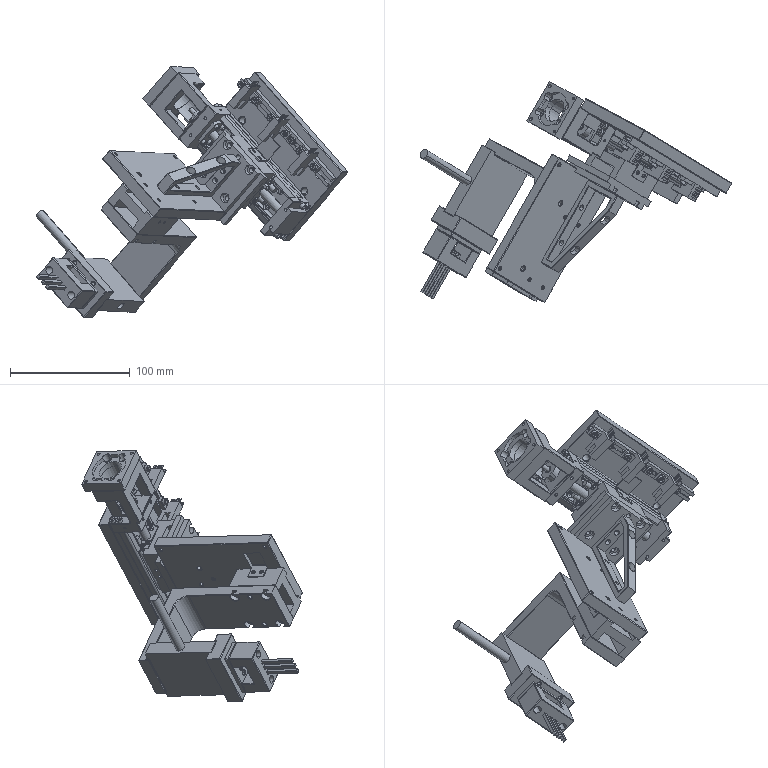Assembly | SolidWorks | mm | 37 component files | 37 solids | 2007 faces | box 260.89 x 184.6 x 210.11 mm | volume 491742 mm3 | plane 1154 | cylinder 578 | cone 238 | spline 35 | torus 2 | commonest cylinder face diameters 2.5 x74 3 x49 1 x41 4 x38 6.5 x36 3.4 x36 8 x30 3.5 x30
Bill of materials:
1z0-123 | 2 |  | Rectangular block with a raised strip along one top edge and a wide rectangular channel cut through the underside, leaving two end legs; four through holes on the top face and two small holes on one side face.
2z0-123 | 1 |  | L-shaped angle bracket: two flat legs at about 90 degrees with an inside fillet at the bend; each leg has two rows of three holes, and small rectangular notches along the edges.
3z0-123 | 1 |  | Rectangular block with a counterbored central through hole flanked by two smaller holes; one face has a longitudinal groove with a smaller hole and a larger bore, and there are small notches and a shallow rectangular slot.
4z0-123 | 1 |  | C-shaped block (rectangular block with a large rectangular notch cut from one side) with two large round holes and three square openings, shown rotated like diamonds, on the back face, plus smaller round holes on the arm faces.
5z0-123 | 1 |  | Flat rectangular plate with chamfered edges and five holes in a line: two smaller outer holes and three larger inner holes that appear stepped.
6z0-123 | 3 |  | Long square-section bar with a larger square head at one end; edges are chamfered and the head end appears to have a round bore.
7z0-123 | 1 |  | Thick rectangular plate with a scattered pattern of holes of several sizes on the main face, small holes near the corners, and a row of holes on one narrow edge face.
8z0-123 | 1 |  | Square plate with a stepped rebate along one edge, several counterbored holes, plain holes of various sizes, small edge notches, and two small rectangular blocks on the opposite face.
9z0-123 | 1 |  | Open triangular/trapezoidal frame made of rectangular-section members with a chamfered corner; the long sloped member has two large holes, and the other members have smaller holes.
GravitySensorZ0-123 | 1 |  | Rectangular block with a cylindrical rod sticking out from one narrow face, and round holes on two other side faces.
f2z0-123 | 1 |  | Thick square block with a large central through bore, surrounded by a pattern of smaller holes and corner holes; one face has stepped, lobed recesses around the bore.
KK40-100_8z0-123 | 1 |  | Long multi-body assembly: a square end block with a large bore and hole pattern, an open rectangular frame section with a cylindrical body inside, a long body with parallel round rods and a plate, and an end block showing several screw-head-like cylinders.
KK40-A1_1z0-123 | 1 |  | Compact rectangular block-like multi-body unit with parallel cylindrical rods running along its length, a top plate with recessed pads and holes, and pan-head cross-recess screws plus protruding round pins at the end faces.
CB3-6-0710z0-123 | 7 |  | Socket-head cap screw shape: cylindrical head with hexagonal socket recess and a plain cylindrical shank with chamfered end.
CBTN3-0710z0-123 | 6 |  | Hexagonal nut with central through bore and chamfered corners on one or both faces.
EE-SX672-0710z0-123 | 3 |  | U-shaped (slotted) housing with two parallel arms separated by a gap, a perpendicular mounting flange with two through holes, and a row of four thin flat pin-like tabs projecting from one end.
SENA34H-400-V50-W150-X250-Y350-N3.5-0710z0-123 | 1 |  | Long straight prismatic bar with a C/slotted channel cross-section and a small transverse hole near mid-length.
Part7z0-123 | 1 |  | Flat rectangular plate with a pattern of through holes of several sizes, including counterbored holes near corners and smaller holes.
ShadingPlateZ0-123 | 2 |  | Bent sheet-like angle bracket (L-shape) with a rounded bend; one leg has two round through holes, the other leg is plain.
ur3_15-0710z0-123 | 1 |  | Hollow thin-walled cylindrical sleeve with an axial split/overlapping seam, resembling a rolled or slotted tube.
Mates:
1. width | GravitySensorZ0-123-1 face at (-90.302, -65.883, 90.305) dir (-0.6119, 0.3716, 0.6982) | GravitySensorZ0-123-1 face at (-59.217, -84.759, 54.836) dir (0.6119, -0.3716, -0.6982) | 1z0-123-1 face at (-3.382, -95.961, 117.465) dir (0.6119, -0.3716, -0.6982) | 1z0-123-1 face at (-27.859, -81.098, 145.394) dir (-0.6119, 0.3716, 0.6982)
2. coincident | GravitySensorZ0-123-1 face at (-59.217, -84.759, 54.836) dir (-0.4977, -0.867, 0.02519) | 3z0-123-1 face at (-59.279, -84.726, 54.764) dir (0.4977, 0.867, -0.02519)
3. coincident | GravitySensorZ0-123-1 face at (-51.151, -52.012, 80.856) dir (0.6147, -0.3321, 0.7154) | 3z0-123-1 face at (-51.411, -88.977, 63.922) dir (-0.6147, 0.3321, -0.7154)
4. coincident | GravitySensorZ0-123-1 face at (-90.302, -65.883, 90.305) dir (-0.6119, 0.3716, 0.6982) | 3z0-123-1 face at (-94.655, -61.26, 84.03) dir (-0.6119, 0.3716, 0.6982)
5. width | 4z0-123-1 face at (-71.913, -121.978, 71.25) dir (0.6147, -0.3321, 0.7154) | 4z0-123-1 face at (-84.207, -115.336, 56.941) dir (-0.6147, 0.3321, -0.7154) | 3z0-123-1 face at (-94.655, -61.26, 84.03) dir (-0.6147, 0.3321, -0.7154) | 3z0-123-1 face at (-76.214, -71.223, 105.493) dir (0.6147, -0.3321, 0.7154)
6. width | 4z0-123-1 face at (-84.207, -115.336, 56.941) dir (0.6119, -0.3716, -0.6982) | 4z0-123-1 face at (-108.683, -100.473, 84.87) dir (-0.6119, 0.3716, 0.6982) | 3z0-123-1 face at (-94.655, -61.26, 84.03) dir (-0.6119, 0.3716, 0.6982) | 3z0-123-1 face at (-63.57, -80.136, 48.561) dir (0.6119, -0.3716, -0.6982)
7. coincident | 4z0-123-1 face at (-78.851, -91.285, 77.48) dir (0.4977, 0.867, -0.02519) | 5z0-123-1 face at (-78.851, -91.285, 77.48) dir (-0.4977, -0.867, 0.02519)
8. coincident | 4z0-123-1 face at (-84.207, -115.336, 56.941) dir (0.6119, -0.3716, -0.6982) | 5z0-123-1 face at (-58.475, -98.569, 70.57) dir (0.6119, -0.3716, -0.6982)
9. coincident | 4z0-123-1 face at (-84.207, -115.336, 56.941) dir (-0.6147, 0.3321, -0.7154) | 5z0-123-1 face at (-95.245, -77.065, 84.189) dir (-0.6147, 0.3321, -0.7154)
10. coincident | 3z0-123-1 face at (-76.86, -87.817, 77.38) dir (-0.4977, -0.867, 0.02519) | 5z0-123-1 face at (-76.86, -87.817, 77.38) dir (0.4977, 0.867, -0.02519)
11. coincident | 4z0-123-1 face at (-84.851, -102.083, 63.646) dir (0.4977, 0.867, -0.02519) | 6z0-123-1 face at (-88.495, -99.459, 81.972) dir (-0.4977, -0.867, 0.02519)
12. coincident | 6z0-123-1 face at (-108.403, -134.138, 82.98) dir (-0.4977, -0.867, 0.02519) | 6z0-123-2 face at (-104.732, -136.368, 78.79) dir (-0.4977, -0.867, 0.02519)
13. coincident | 6z0-123-1 face at (-108.403, -134.138, 82.98) dir (-0.4977, -0.867, 0.02519) | 6z0-123-3 face at (-101.06, -138.597, 74.601) dir (-0.4977, -0.867, 0.02519)
14. concentric | 5z0-123-1 face at (-77.855, -89.551, 77.43) dir (-0.4977, -0.867, 0.02519) r 2.1 | 6z0-123-2 face at (-83.828, -99.955, 77.732) dir (0.4977, 0.867, -0.02519) r 2.1
15. concentric | 5z0-123-1 face at (-74.184, -91.78, 73.241) dir (-0.4977, -0.867, 0.02519) r 2.1 | 6z0-123-3 face at (-80.156, -102.184, 73.543) dir (0.4977, 0.867, -0.02519) r 2.1
16. concentric | 6z0-123-1 face at (-87.499, -97.725, 81.922) dir (0.4977, 0.867, -0.02519) r 2.1 | ur3_15-0710z0-123-1 face at (-83.767, -91.223, 81.733) dir (-0.4977, -0.867, 0.02519) r 1.5
17. tangent | 6z0-123-1 face at (-87.499, -97.725, 81.922) dir (0.4977, 0.867, -0.02519) | ur3_15-0710z0-123-1 face at (-87.969, -97.077, 83.049) dir (1, 0, 0)
18. coincident | 7z0-123-1 face at (-0.3267, -18.072, 178.948) dir (0.4977, 0.867, -0.02519) | 8z0-123-1 face at (43.801, -43.838, 164.019) dir (-0.4977, -0.867, 0.02519)
19. coincident | 8z0-123-1 face at (42.307, -46.439, 164.094) dir (-0.4977, -0.867, 0.02519) | 9z0-123-1 face at (36.147, -43.316, 149.872) dir (0.4977, 0.867, -0.02519)
20. coincident | 7z0-123-1 face at (-0.1369, -82.082, 163.051) dir (0.6147, -0.3321, 0.7154) | 9z0-123-1 face at (-3.67, -112.674, 151.887) dir (-0.6147, 0.3321, -0.7154)
21. width | 9z0-123-1 face at (28.532, -84.637, 165.188) dir (0.6119, -0.3716, -0.6982) | 9z0-123-1 face at (22.413, -80.921, 172.17) dir (-0.6119, 0.3716, 0.6982) | 8z0-123-1 face at (37.941, -45.023, 126.572) dir (0.6119, -0.3716, -0.6982) | 8z0-123-1 face at (9.793, -27.93, 158.69) dir (-0.6119, 0.3716, 0.6982)
22. coincident | 1z0-123-1 face at (-26.819, -108.037, 131.996) dir (-0.6147, 0.3321, -0.7154) | 2z0-123-1 face at (23.992, -48.278, 116.08) dir (0.6147, -0.3321, 0.7154)
23. concentric | 1z0-123-1 face at (-16.722, -114.168, 120.476) dir (-0.6147, 0.3321, -0.7154) r 2 | 2z0-123-1 face at (-22.869, -110.847, 113.321) dir (-0.6147, 0.3321, -0.7154) r 2
24. coincident | 1z0-123-1 face at (-3.382, -95.961, 117.465) dir (0.6119, -0.3716, -0.6982) | 2z0-123-1 face at (-27.018, -77.512, 86.933) dir (0.6119, -0.3716, -0.6982)
25. coincident | GravitySensorZ0-123-1 face at (-27.613, -29.706, 53.236) dir (0.4977, 0.867, -0.02519) | 2z0-123-1 face at (-47.587, -17.054, 94.021) dir (-0.4977, -0.867, 0.02519)
26. concentric | 7z0-123-1 face at (28.447, -35.339, 153.201) dir (0.4977, 0.867, -0.02519) r 2 | 8z0-123-1 face at (28.447, -35.339, 153.201) dir (-0.4977, -0.867, 0.02519) r 2
27. concentric | 7z0-123-1 face at (34.566, -39.054, 146.219) dir (0.4977, 0.867, -0.02519) r 2 | 8z0-123-1 face at (34.566, -39.054, 146.219) dir (-0.4977, -0.867, 0.02519) r 2
28. coincident | KK40-100A1-F0z0-123-2/KK40-A1_1z0-123-1 face at (64.552, -28.453, 150.815) dir (-0.4977, -0.867, 0.02519) | 1z0-123-2 face at (61.893, -26.352, 170.569) dir (0.4977, 0.867, -0.02519)
29. coincident | KK40-100A1-F0z0-123-2/KK40-A1_1z0-123-1 face at (85.864, -35.462, 163.914) dir (0.6147, -0.3321, 0.7154) | 1z0-123-2 face at (83.652, -39.029, 164.16) dir (-0.6147, 0.3321, -0.7154)
30. coincident | KK40-100A1-F0z0-123-2/KK40-A1_1z0-123-1 face at (75.144, -20.462, 146.822) dir (0.6119, -0.3716, -0.6982) | 1z0-123-2 face at (79.493, -56.093, 169.596) dir (0.6119, -0.3716, -0.6982)
31. coincident | 8z0-123-1 face at (74.822, -64.948, 169.499) dir (0.6147, -0.3321, 0.7154) | 1z0-123-2 face at (79.493, -56.093, 169.596) dir (0.6147, -0.3321, 0.7154)
32. width | 8z0-123-1 face at (64.418, -48.174, 144.293) dir (0.6119, -0.3716, -0.6982) | 8z0-123-1 face at (30.151, -27.365, 183.392) dir (-0.6119, 0.3716, 0.6982) | 1z0-123-2 face at (51.957, -39.372, 201.016) dir (-0.6119, 0.3716, 0.6982) | 1z0-123-2 face at (79.493, -56.093, 169.596) dir (0.6119, -0.3716, -0.6982)
33. coincident | KK40-100A1-F0z0-123-2/KK40-100_8z0-123-1 face at (152.075, -58.532, 50.893) dir (0.4977, 0.867, -0.02519) | Part7z0-123-1 face at (84.569, -15.914, 183.885) dir (-0.4977, -0.867, 0.02519)
34. coincident | KK40-100A1-F0z0-123-2/KK40-100_8z0-123-1 face at (83.132, -48.833, 114.21) dir (0.6119, -0.3716, -0.6982) | Part7z0-123-1 face at (96.696, -24.925, 113.375) dir (0.6119, -0.3716, -0.6982)
35. coincident | KK40-100A1-F0z0-123-2/KK40-100_8z0-123-1 face at (151.519, -58.8, 50.548) dir (-0.6147, 0.3321, -0.7154) | Part7z0-123-1 face at (23.267, 19.664, 197.16) dir (-0.6147, 0.3321, -0.7154)
36. coincident | 8z0-123-1 face at (47.285, -37.769, 163.843) dir (0.4977, 0.867, -0.02519) | 1z0-123-2 face at (53.431, -41.09, 170.997) dir (-0.4977, -0.867, 0.02519)
37. coincident | Part7z0-123-1 face at (84.569, -15.914, 183.885) dir (-0.4977, -0.867, 0.02519) | KKSwitch-0710z0-123-1/SENA34H-400-V50-W150-X250-Y350-N3.5-0710z0-123-1 face at (67.524, -4.247, 248.672) dir (0.4977, 0.867, -0.02519)
38. coincident | Part7z0-123-1 face at (23.267, 19.664, 197.16) dir (-0.6119, 0.3716, 0.6982) | KKSwitch-0710z0-123-1/SENA34H-400-V50-W150-X250-Y350-N3.5-0710z0-123-1 face at (59.006, -6.46, 242.384) dir (-0.6119, 0.3716, 0.6982)
39. coincident | 1z0-123-2 face at (79.493, -56.093, 169.596) dir (0.6147, -0.3321, 0.7154) | ShadingPlateZ0-123-1 face at (74.243, -33.613, 184.541) dir (-0.6147, 0.3321, -0.7154)
40. concentric | 1z0-123-2 face at (75.945, -36.4, 181.786) dir (0.6147, -0.3321, 0.7154) r 1.25 | ShadingPlateZ0-123-1 face at (75.945, -36.4, 181.786) dir (0.6147, -0.3321, 0.7154) r 1.75
41. concentric | 1z0-123-2 face at (71.049, -33.427, 187.372) dir (0.6147, -0.3321, 0.7154) r 1.25 | ShadingPlateZ0-123-1 face at (71.049, -33.427, 187.372) dir (0.6147, -0.3321, 0.7154) r 1.75
42. parallel | 4z0-123-1 face at (-80.691, -90.229, 77.455) dir (0.6119, -0.3716, -0.6982) | 6z0-123-2 face at (-102.892, -137.423, 78.816) dir (0.6119, -0.3716, -0.6982)
43. parallel | 4z0-123-1 face at (-75.183, -93.573, 71.171) dir (0.6147, -0.3321, 0.7154) | 6z0-123-3 face at (-101.056, -138.538, 76.722) dir (0.6147, -0.3321, 0.7154)
44. concentric | 5z0-123-1 face at (-81.527, -87.321, 81.619) dir (-0.4977, -0.867, 0.02519) r 2.1 | ur3_15-0710z0-123-1 face at (-83.767, -91.223, 81.733) dir (-0.4977, -0.867, 0.02519) r 1.5
45. parallel | 4z0-123-1 face at (-82.526, -89.115, 79.549) dir (-0.6119, 0.3716, 0.6982) | 6z0-123-1 face at (-110.243, -133.083, 82.954) dir (-0.6119, 0.3716, 0.6982)
46. coincident | 1z0-123-1 face at (-27.859, -81.098, 145.394) dir (-0.6119, 0.3716, 0.6982) | ShadingPlateZ0-123-2 face at (-28.666, -105.651, 157.753) dir (0.6119, -0.3716, -0.6982)
47. concentric | 1z0-123-1 face at (-27.597, -101.685, 156.579) dir (-0.6119, 0.3716, 0.6982) r 1.25 | ShadingPlateZ0-123-2 face at (-27.597, -101.685, 156.579) dir (-0.6119, 0.3716, 0.6982) r 1.75
48. concentric | 1z0-123-1 face at (-31.579, -108.621, 156.78) dir (-0.6119, 0.3716, 0.6982) r 1.25 | ShadingPlateZ0-123-2 face at (-31.579, -108.621, 156.78) dir (-0.6119, 0.3716, 0.6982) r 1.75
49. distance | KKSwitch-0710z0-123-1/SENA34H-400-V50-W150-X250-Y350-N3.5-0710z0-123-1 face at (64.538, -9.449, 248.823) dir (0.6147, -0.3321, 0.7154) | Part7z0-123-1 face at (72.442, -6.904, 254.396) dir (0.6147, -0.3321, 0.7154)
50. concentric | 1z0-123-1 face at (-37.303, -113.362, 138.532) dir (-0.6147, 0.3321, -0.7154) r 3.25 | 7z0-123-1 face at (-25.009, -120.004, 152.841) dir (-0.6147, 0.3321, -0.7154) r 1.25
51. coincident | 1z0-123-1 face at (-14.525, -114.679, 146.305) dir (0.6147, -0.3321, 0.7154) | 7z0-123-1 face at (-6.284, -78.761, 155.897) dir (-0.6147, 0.3321, -0.7154)
52. concentric | KK40-100_8z0-123-1 face at (12, 13, 0) dir (1, 0, 0) r 10 | KK40-100A1-F0z0-123 face at (32.5, 13, 0) dir (1, 0, 0) r 15
53. coincident | KK40-100A1-F0z0-123 face at (57.5, -3, 16) dir (-1, 0, 0) | f2z0-123-1 face at (57.5, 13, 0) dir (1, 0, 0)
54. concentric | KK40-100A1-F0z0-123 face at (32.5, 13, 0) dir (1, 0, 0) r 15 | f2z0-123-1 face at (49, 13, 0) dir (1, 0, 0) r 10
55. coincident | KK40-100A1-F0z0-123 face at (57.5, -6, -16) dir (0, -1, 0) | f2z0-123-1 face at (57.5, -6, 19) dir (0, -1, 0)
56. coincident | KK40-100_8z0-123-1 face at (49, 30, -19.8) dir (1, 0, 0) | f2z0-123-1 face at (49, 13, 0) dir (-1, 0, 0)
57. parallel | KK40-100_8z0-123-1 face at (49, 0.5, -19.8) dir (0, -1, 0) | f2z0-123-1 face at (57.5, -6, 19) dir (0, -1, 0)
58. width | CBTN3-0710z0-123-1 face at (1.663, -3.194, 216.912) dir (0, -1, 0) | CBTN3-0710z0-123-1 face at (1.663, 2.306, 220.088) dir (0, 1, 0) | SENA34H-400-V50-W150-X250-Y350-N3.5-0710z0-123-1 face at (-0.7374, 2.406, 320) dir (0, -1, 0) | SENA34H-400-V50-W150-X250-Y350-N3.5-0710z0-123-1 face at (2.263, -3.294, 320) dir (0, 1, 0)
59. coincident | SENA34H-400-V50-W150-X250-Y350-N3.5-0710z0-123-1 face at (-0.7374, 1.256, 320) dir (1, 0, 0) | CBTN3-0710z0-123-1 face at (-0.7374, 0.5263, 217.94) dir (-1, 0, 0)
60. concentric | CB3-6-0710z0-123-1 face at (-2.391, -0.4437, 218.5) dir (1, 0, 0) r 1.5 | CBTN3-0710z0-123-1 face at (0.4626, -0.4437, 218.5) dir (1, 0, 0) r 1.193
61. coincident | SENA34H-400-V50-W150-X250-Y350-N3.5-0710z0-123-1 face at (-2.237, -2.144, 320) dir (-1, 0, 0) | EE-SX672-0710z0-123-1 face at (-2.237, 15.456, 231.2) dir (1, 0, 0)
62. concentric | CB3-6-0710z0-123-1 face at (-2.391, -0.4437, 218.5) dir (1, 0, 0) r 1.5 | EE-SX672-0710z0-123-1 face at (-5.237, -0.4437, 218.5) dir (-1, 0, 0) r 1.6
63. width | CBTN3-0710z0-123-9 face at (1.663, -3.194, 235.912) dir (0, -1, 0) | CBTN3-0710z0-123-9 face at (1.663, 2.306, 239.088) dir (0, 1, 0) | SENA34H-400-V50-W150-X250-Y350-N3.5-0710z0-123-1 face at (2.263, -3.294, 320) dir (0, 1, 0) | SENA34H-400-V50-W150-X250-Y350-N3.5-0710z0-123-1 face at (-0.7374, 2.406, 320) dir (0, -1, 0)
64. coincident | SENA34H-400-V50-W150-X250-Y350-N3.5-0710z0-123-1 face at (-0.7374, -3.294, 320) dir (1, 0, 0) | CBTN3-0710z0-123-9 face at (-0.7374, 0.5263, 236.94) dir (-1, 0, 0)
65. concentric | CB3-6-0710z0-123-13 face at (-2.391, -0.4437, 237.5) dir (1, 0, 0) r 1.5 | CBTN3-0710z0-123-9 face at (0.4626, -0.4437, 237.5) dir (1, 0, 0) r 1.193
66. coincident | EE-SX672-0710z0-123-1 face at (-5.237, -3.544, 241) dir (-1, 0, 0) | CB3-6-0710z0-123-13 face at (-5.237, -0.4248, 239.625) dir (1, 0, 0)
67. concentric | EE-SX672-0710z0-123-1 face at (-5.237, -0.4437, 237.5) dir (-1, 0, 0) r 1.6 | CB3-6-0710z0-123-13 face at (-2.391, -0.4437, 237.5) dir (1, 0, 0) r 1.5
68. coincident | CB3-6-0710z0-123-1 face at (-5.237, 1.655, 218.832) dir (1, 0, 0) | EE-SX672-0710z0-123-1 face at (-5.237, 2.656, 215) dir (-1, 0, 0)
69. concentric | SENA34H-400-V50-W150-X250-Y350-N3.5-0710z0-123-1 face at (3.763, -0.4437, 250) dir (-1, 0, 0) r 1.75 | CB3-6-0710z0-123-16 face at (0.609, -0.4437, 250) dir (1, 0, 0) r 1.5
70. coincident | SENA34H-400-V50-W150-X250-Y350-N3.5-0710z0-123-1 face at (-2.237, 4.056, 320) dir (-1, 0, 0) | CB3-6-0710z0-123-16 face at (-2.237, -0.4248, 252.125) dir (1, 0, 0)
71. distance | EE-SX672-0710z0-123-1 face at (-5.237, 2.656, 215) dir (0, 0, -1) | SENA34H-400-V50-W150-X250-Y350-N3.5-0710z0-123-1 face at (-2.237, 4.056, 200) dir (0, 0, -1)